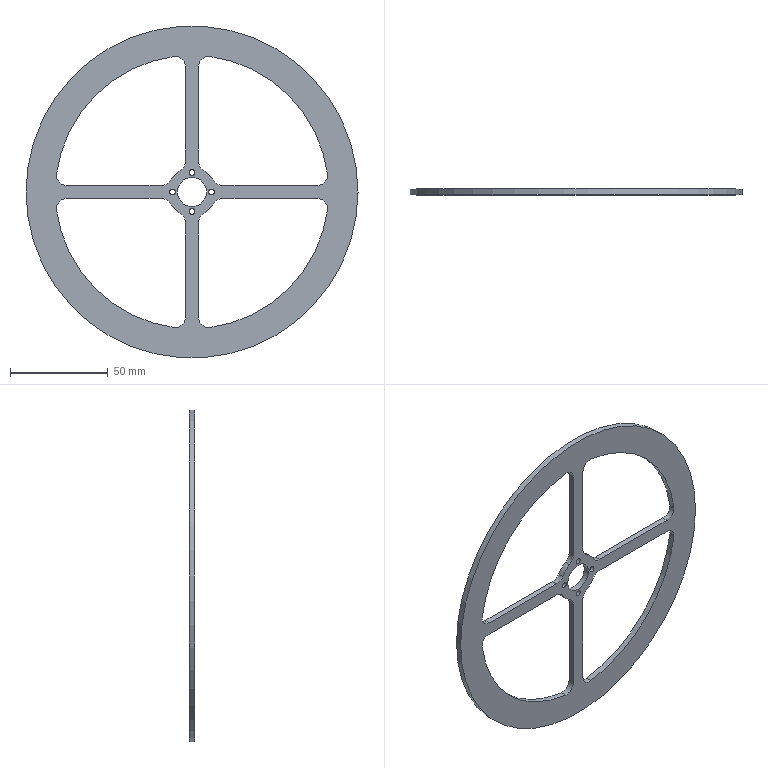Component | NX | WHEEL | 1 solid | 40 faces | volume 27816 mm3 | cylinder 30 | plane 10 | commonest cylinder face diameters 10 x16 140 x4 25 x4 3 x4 15 x1 170 x1